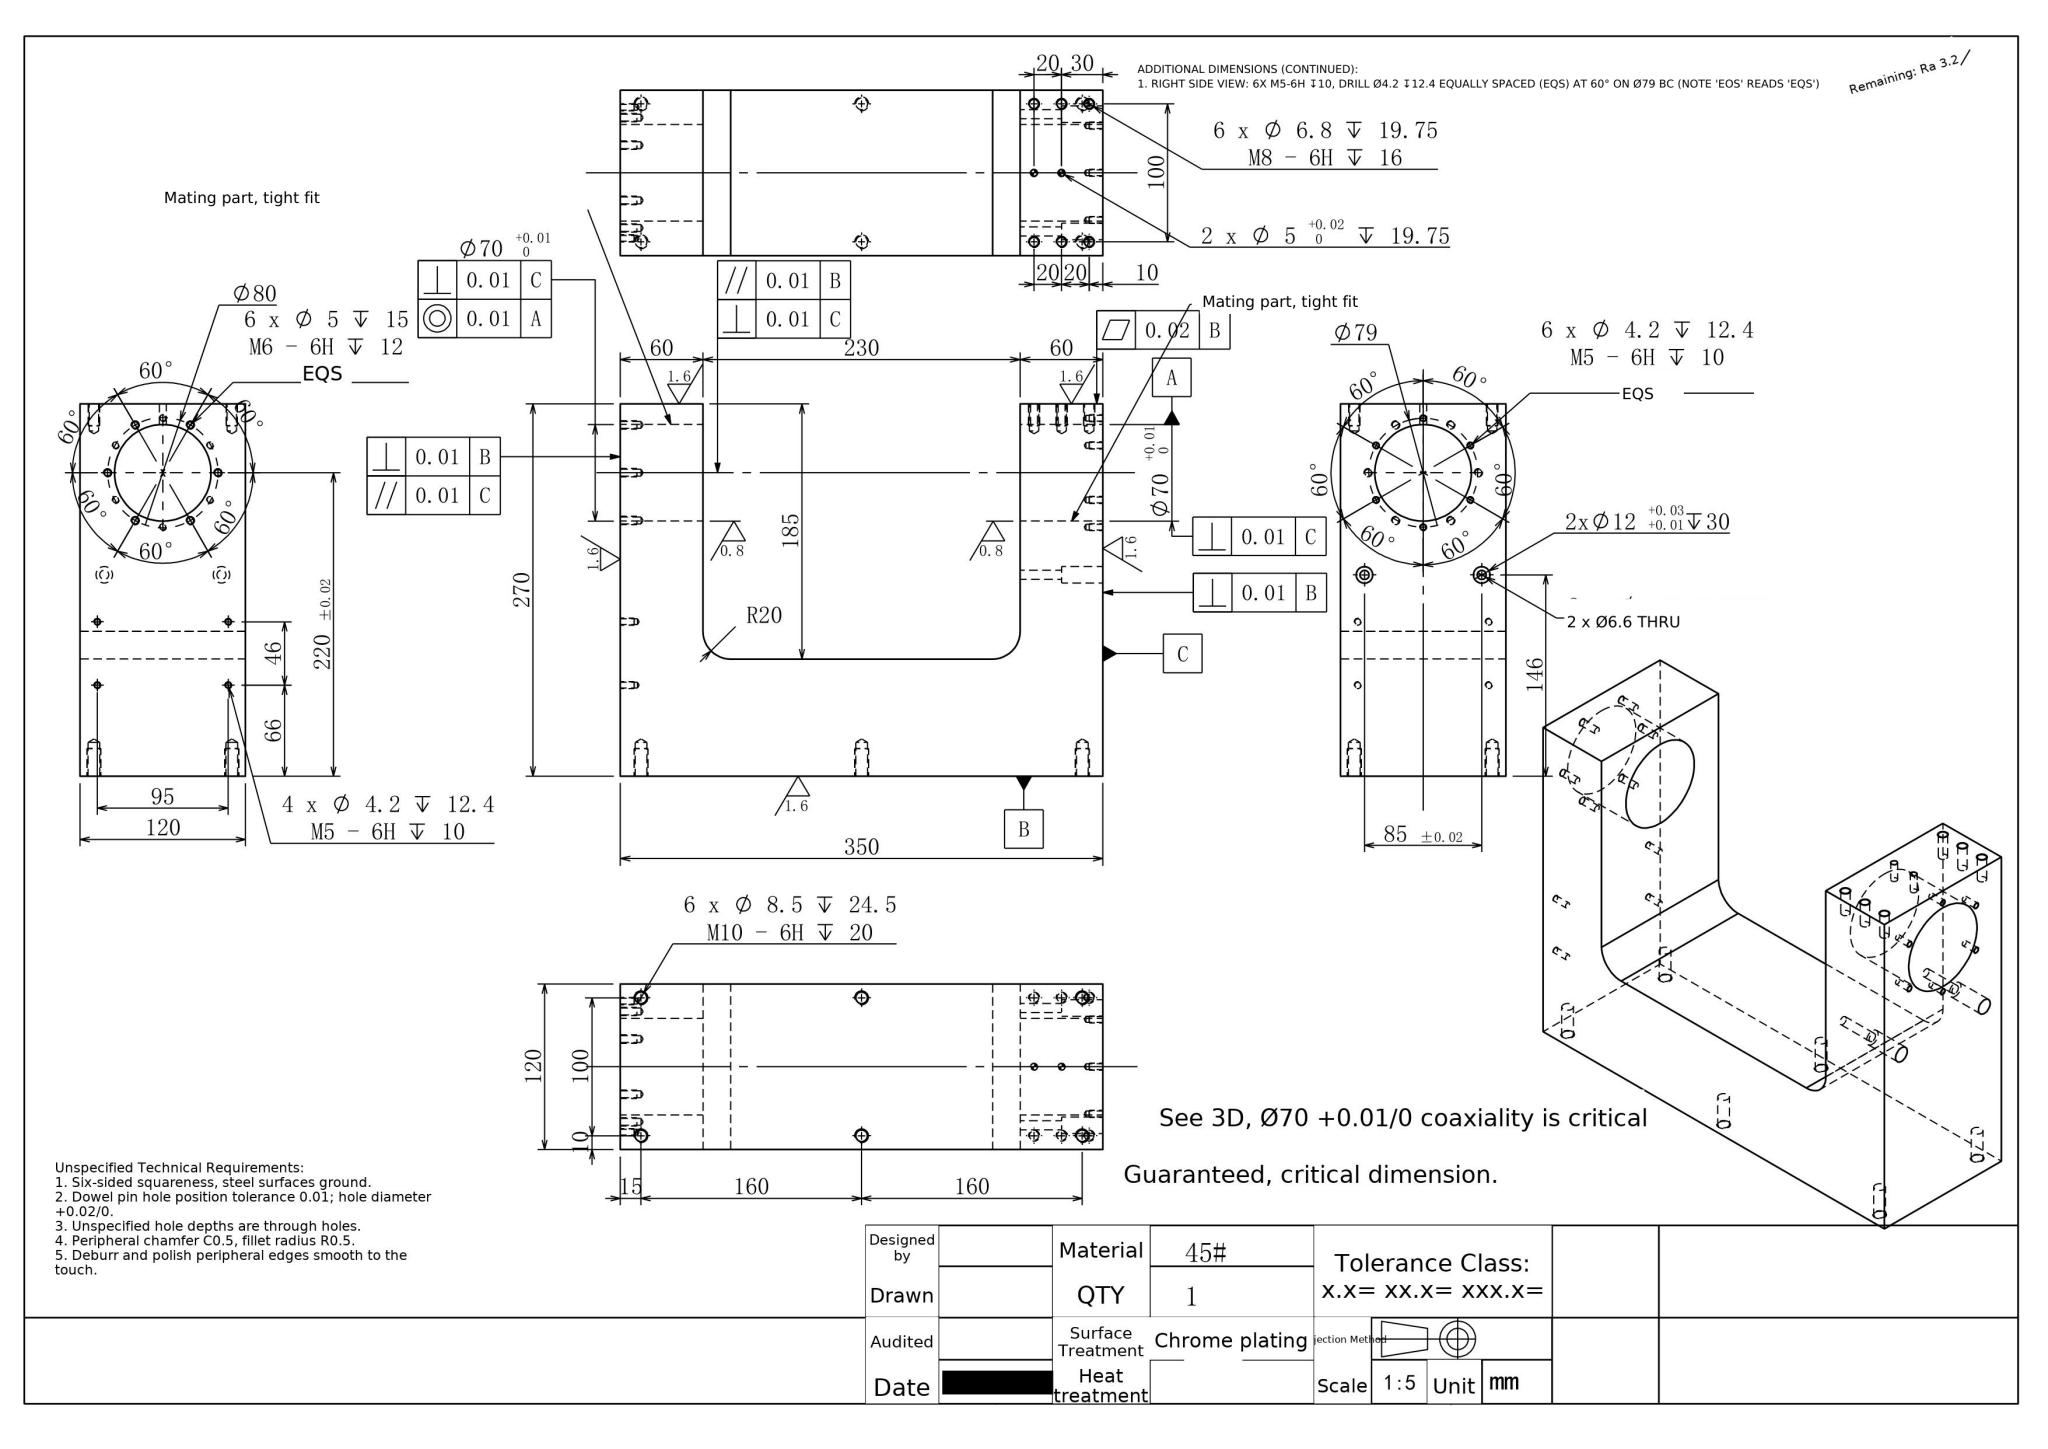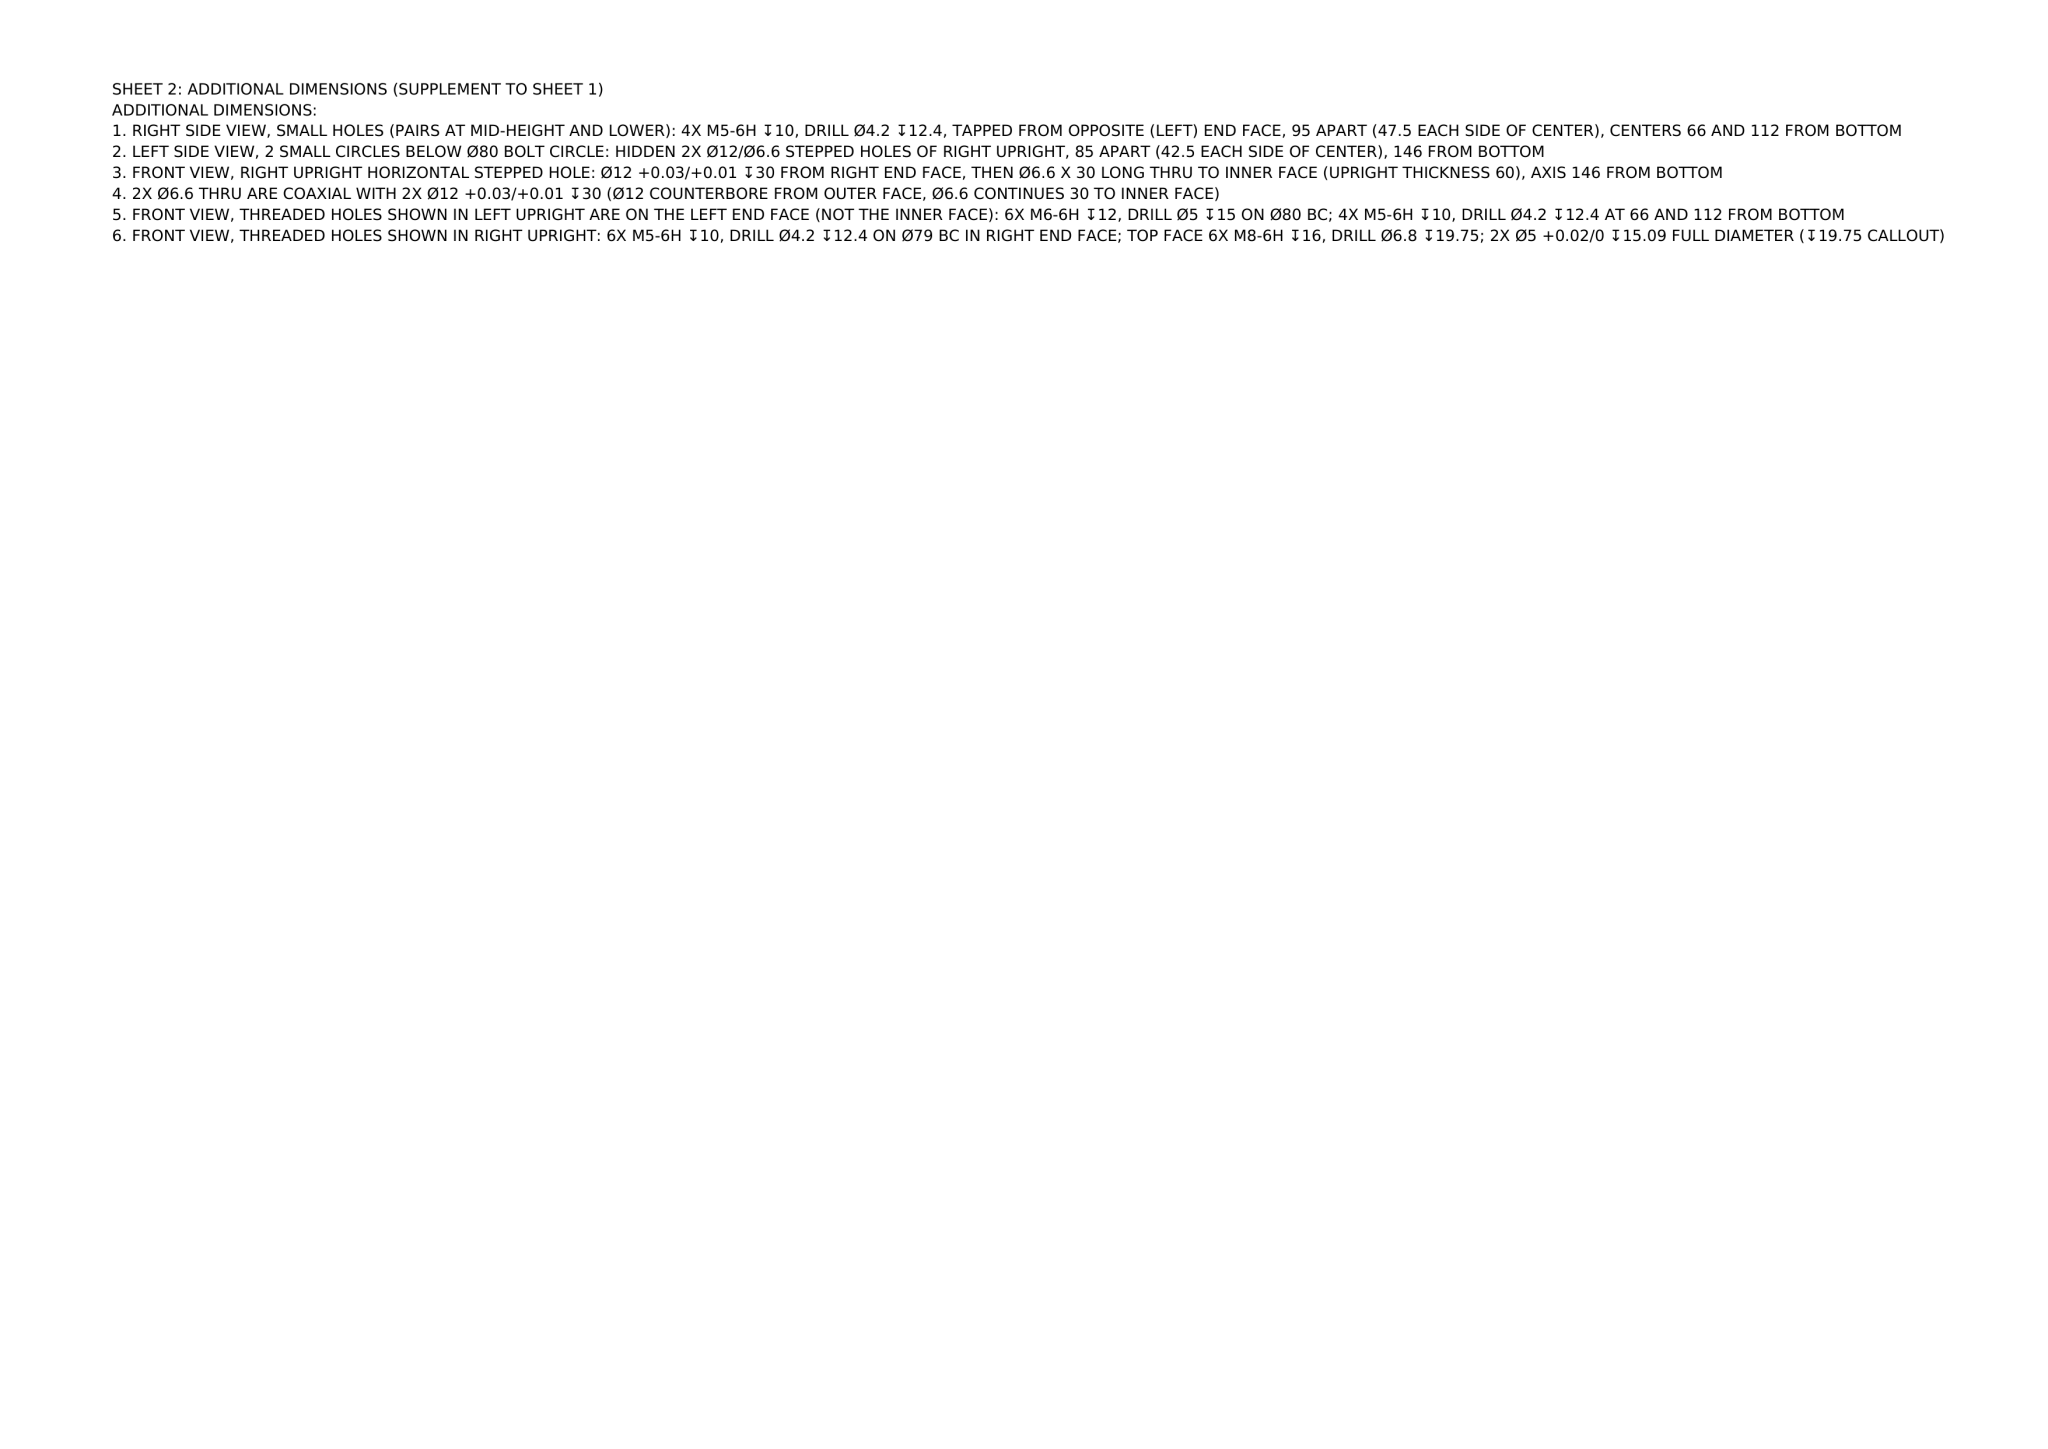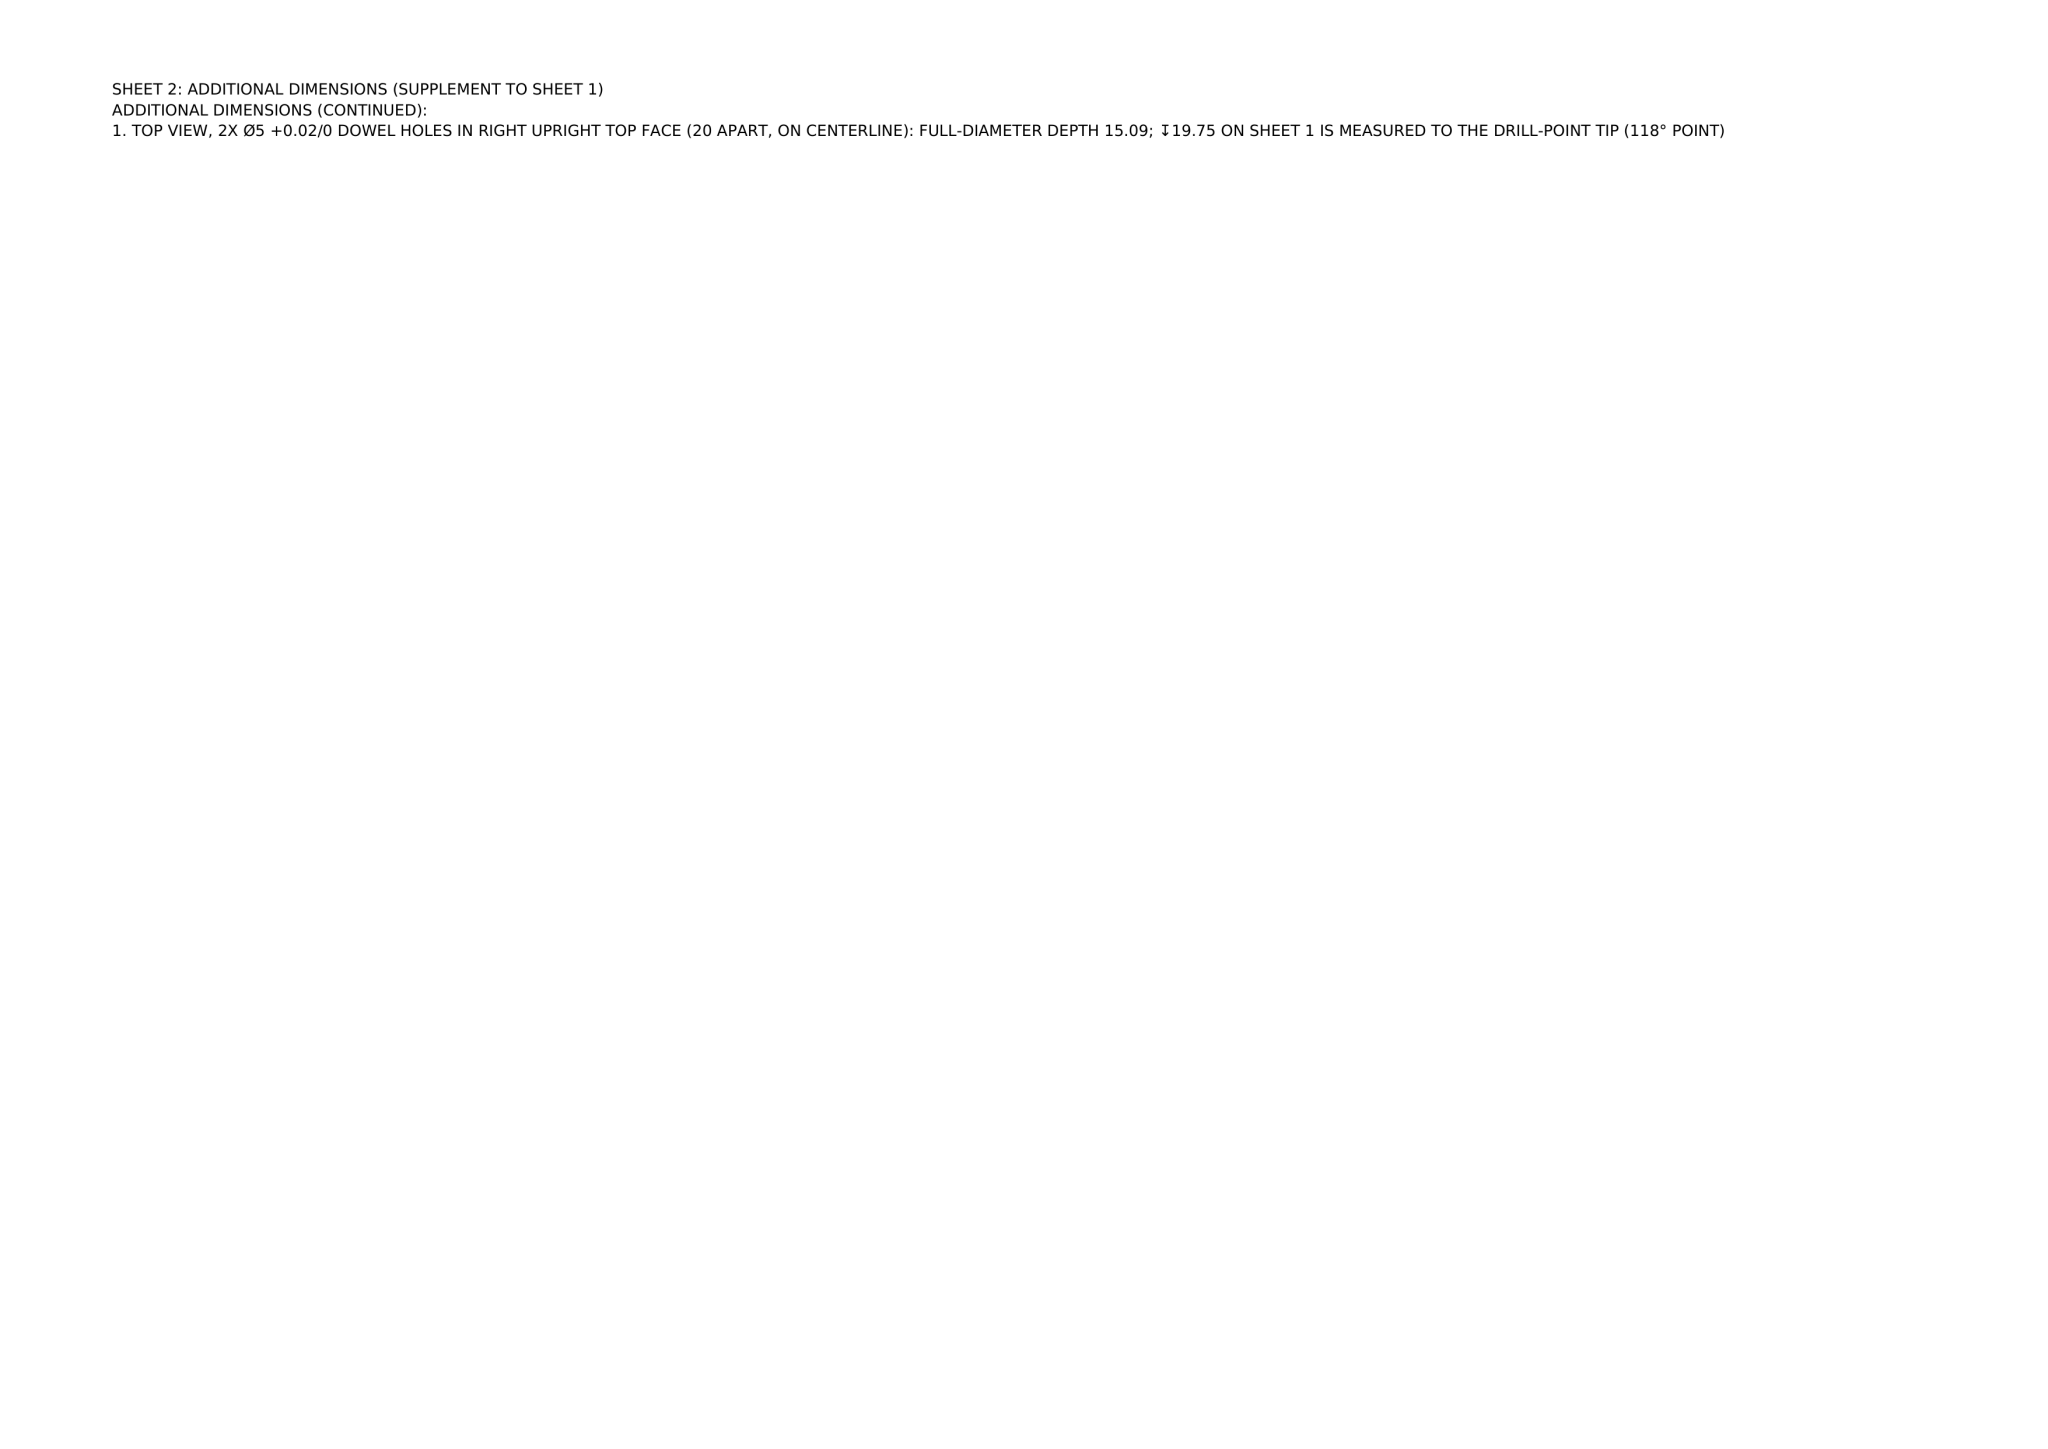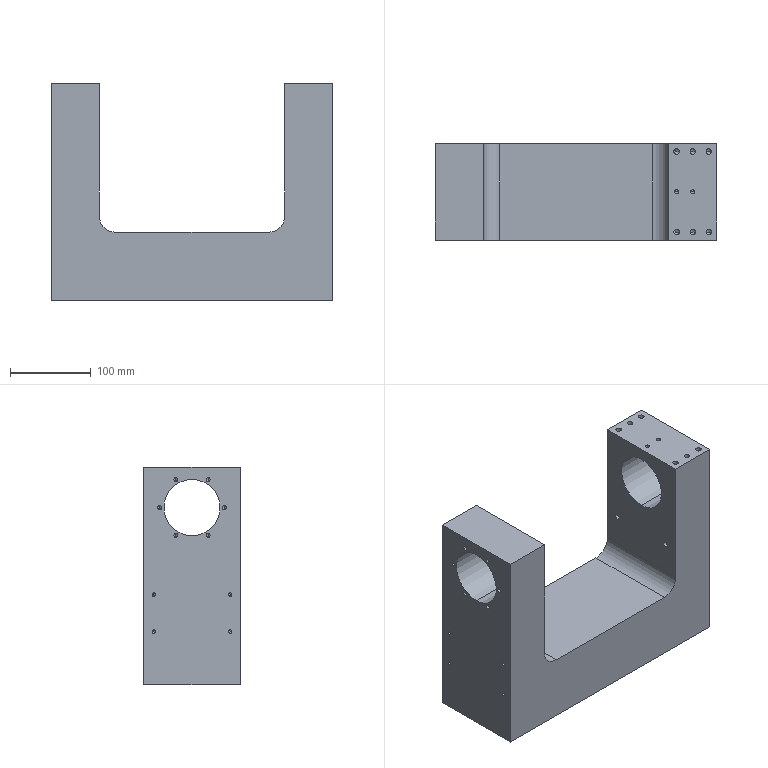Part | NX | mm | 1 solid | 142 faces | box 350 x 120 x 270 mm | volume 5766674 mm3 | cylinder 74 | cone 56 | plane 12 | commonest cylinder face diameters 4.2 x20 5 x16 8.5 x12 6.8 x12 12 x4 70 x4 6.6 x4 40 x2